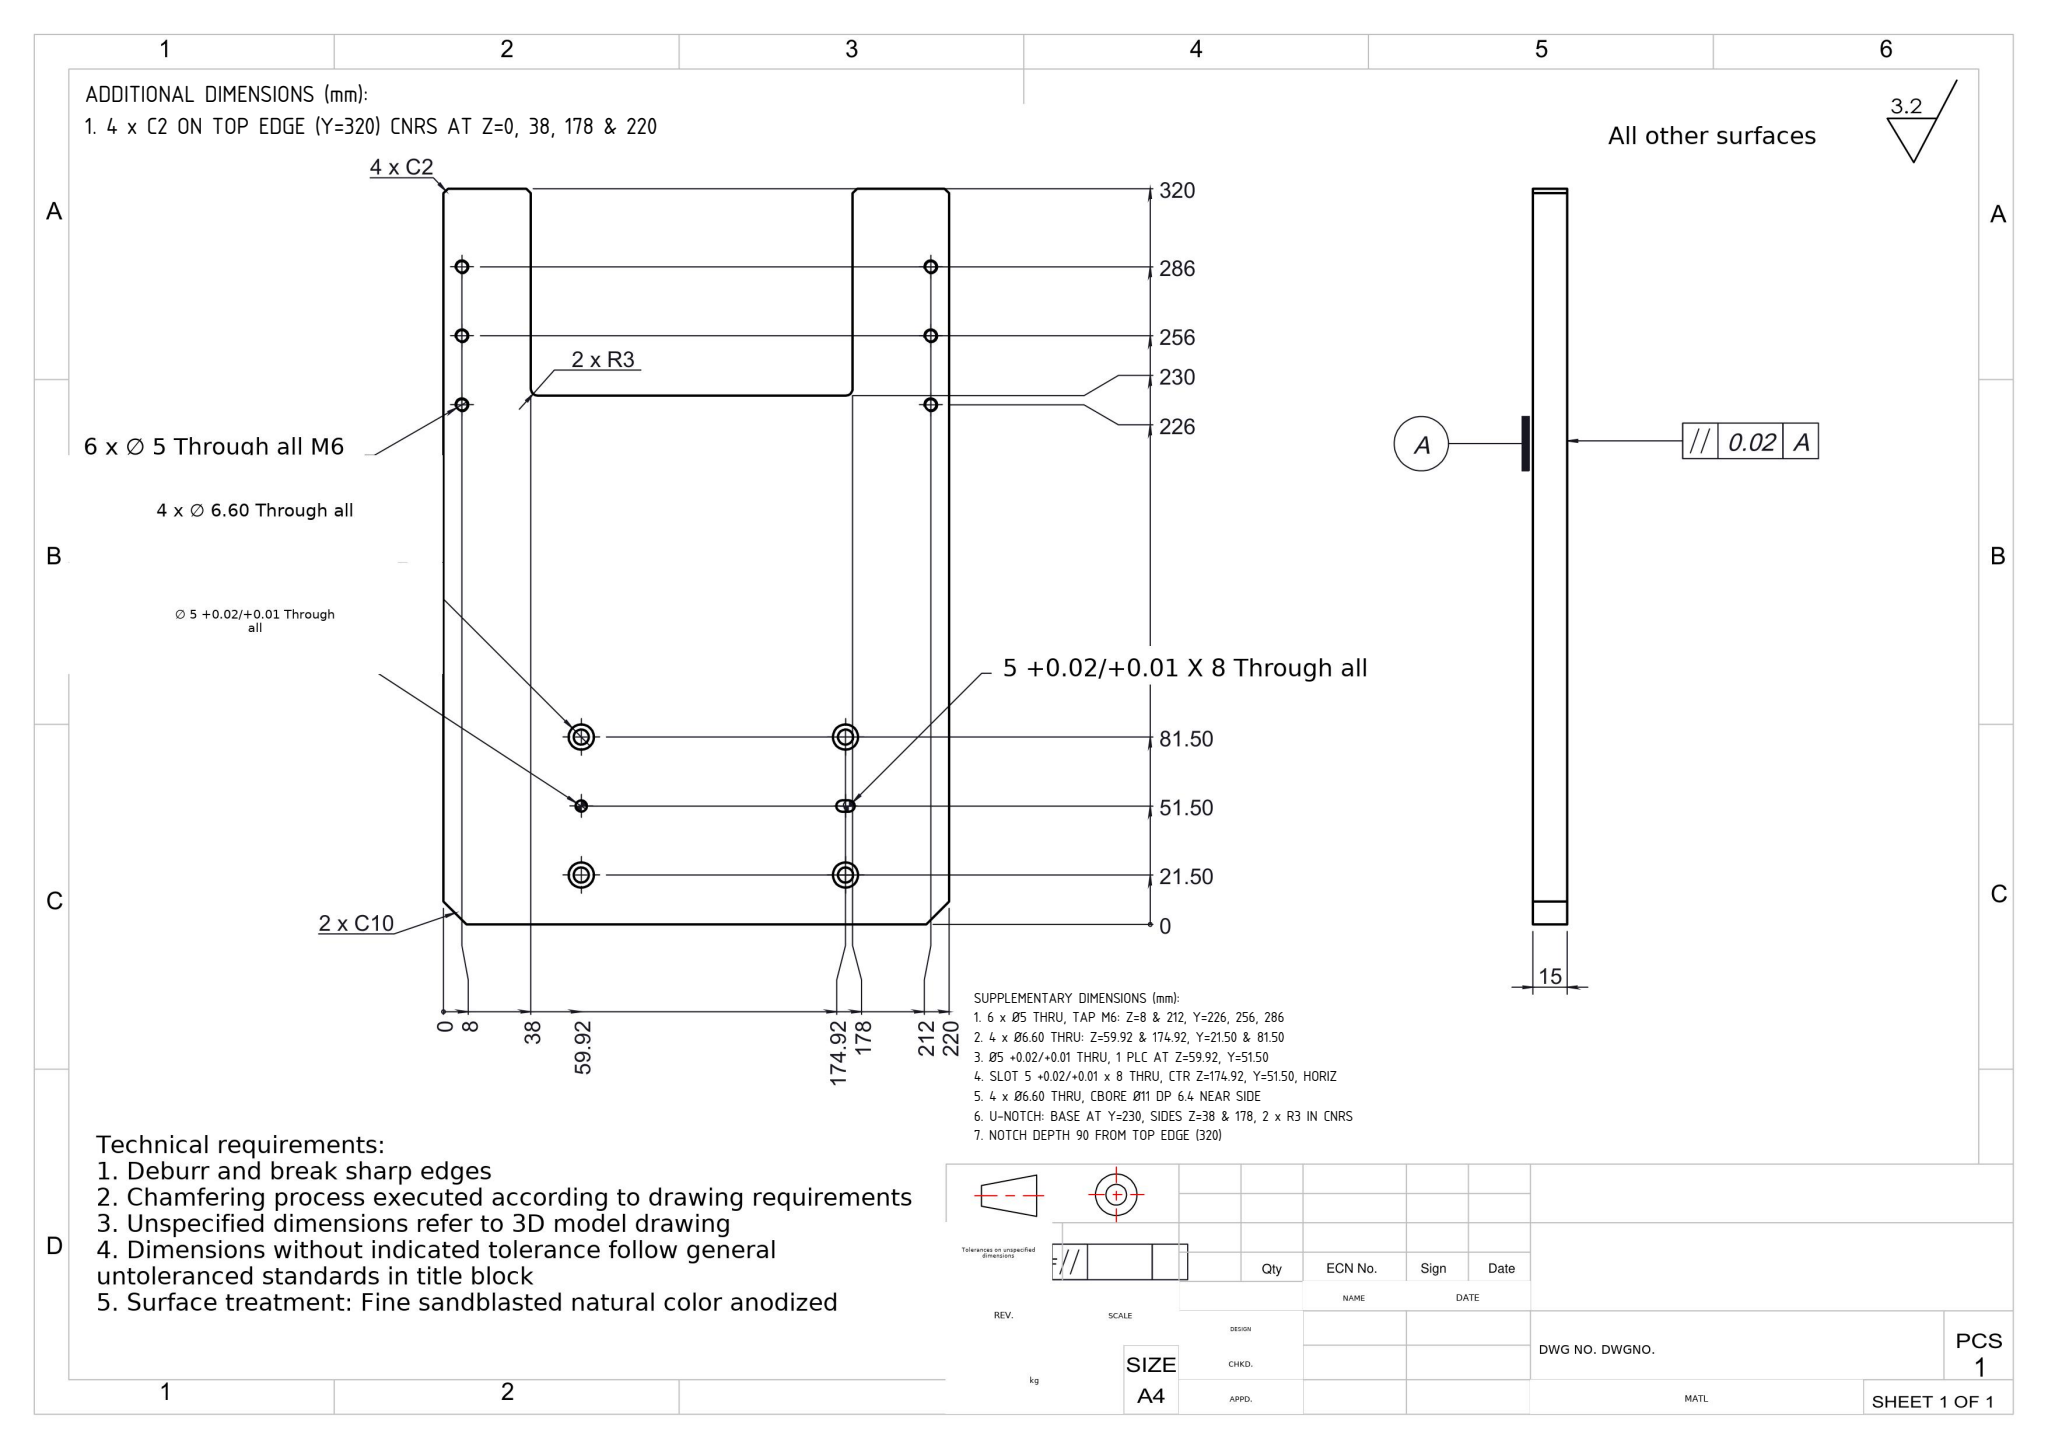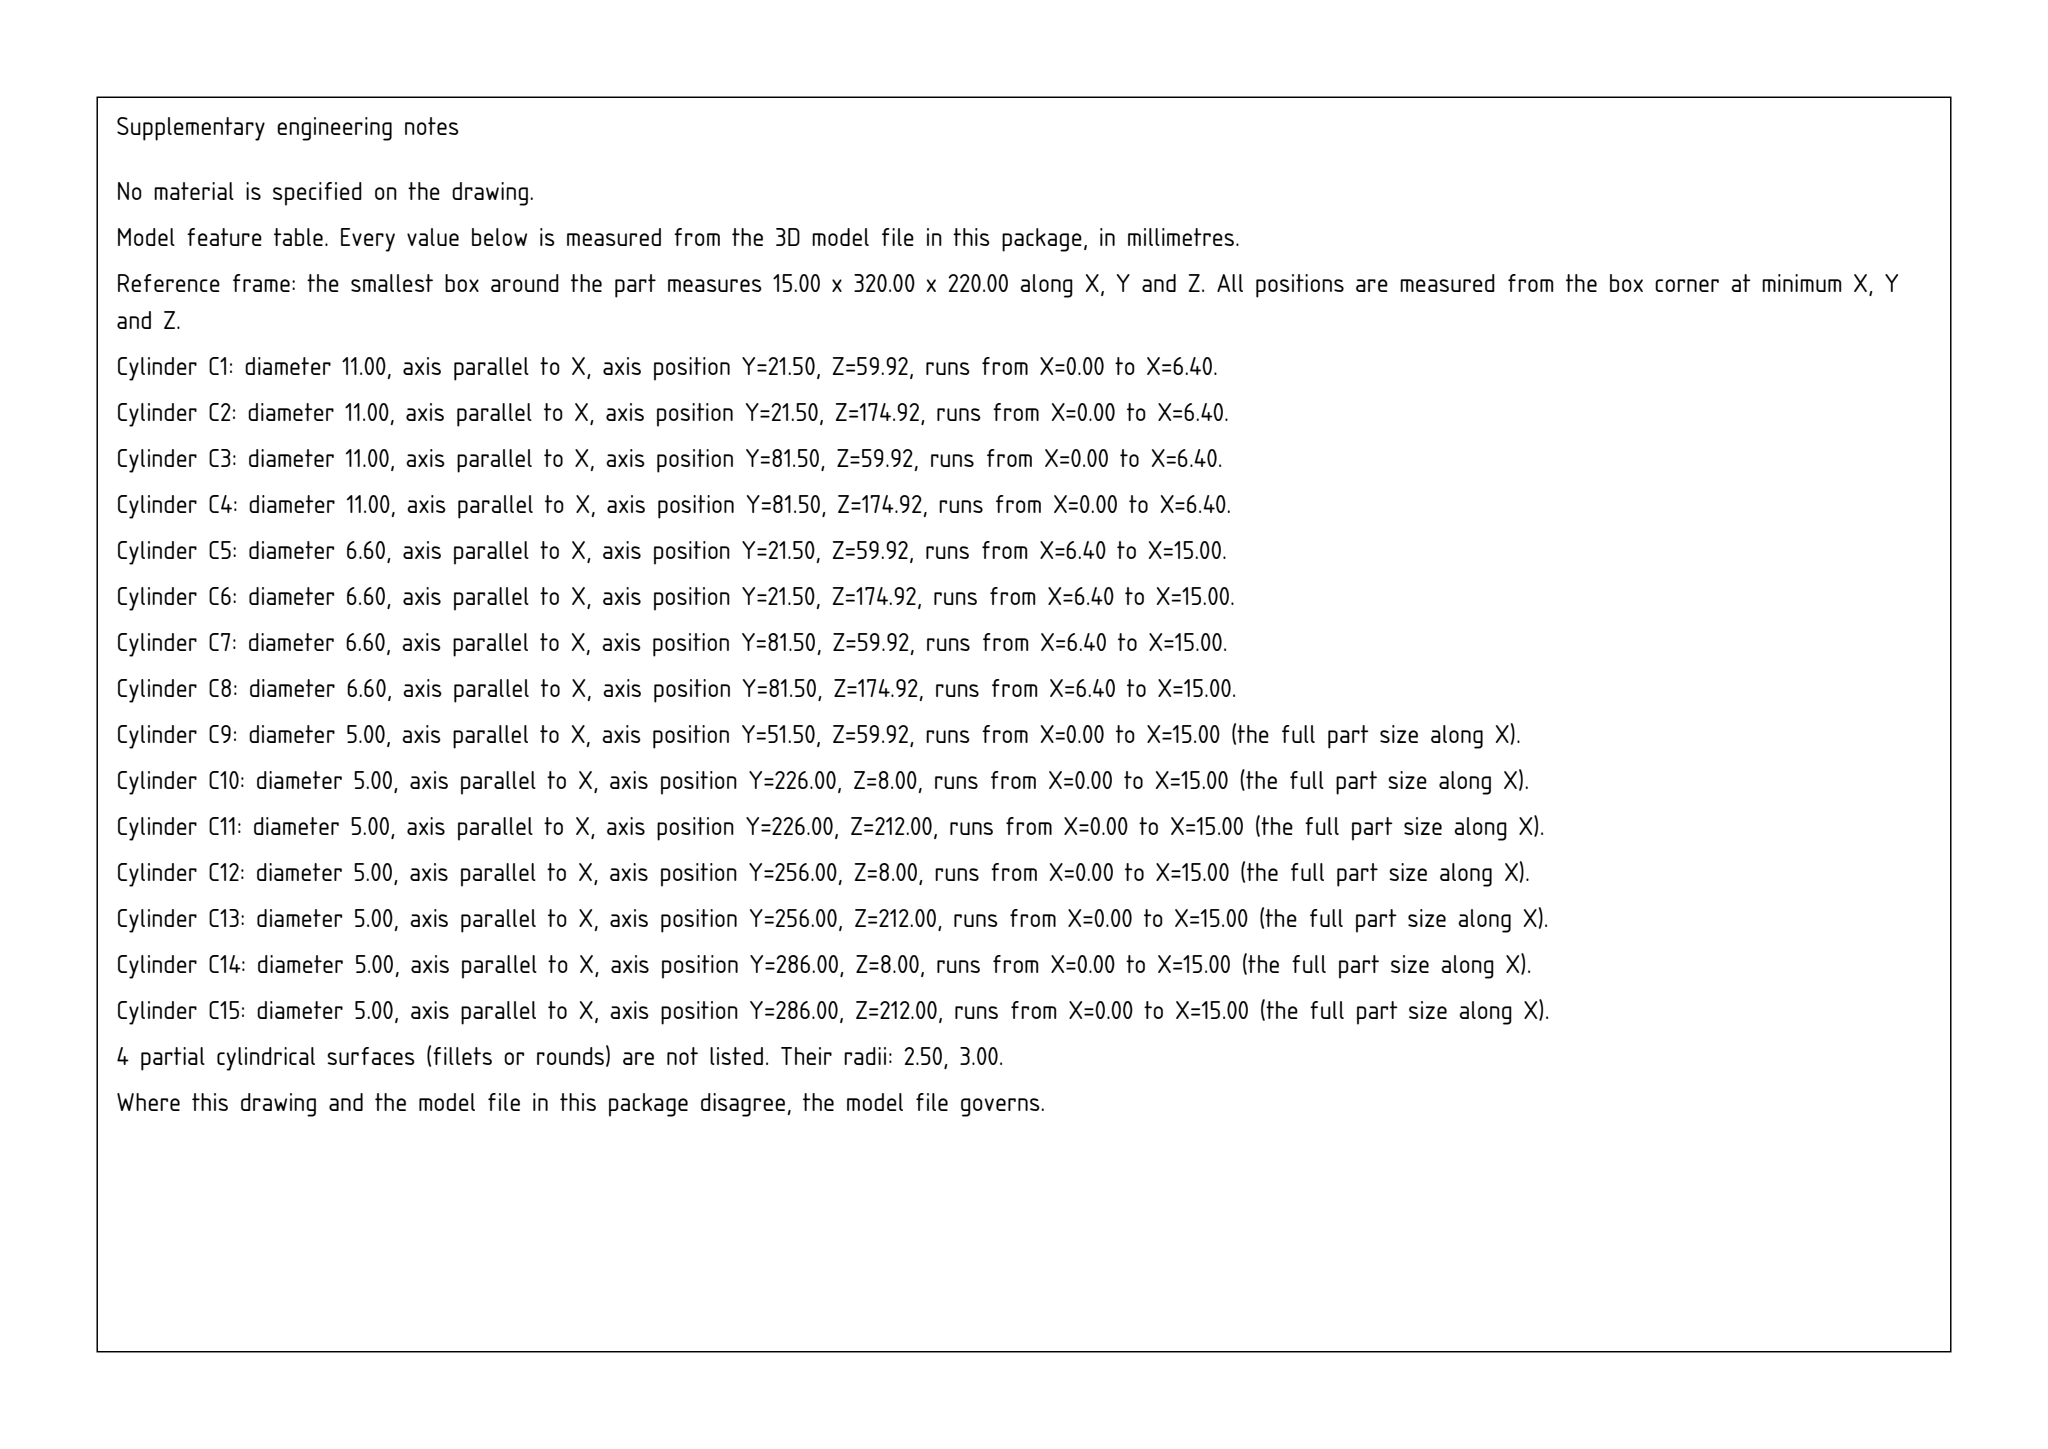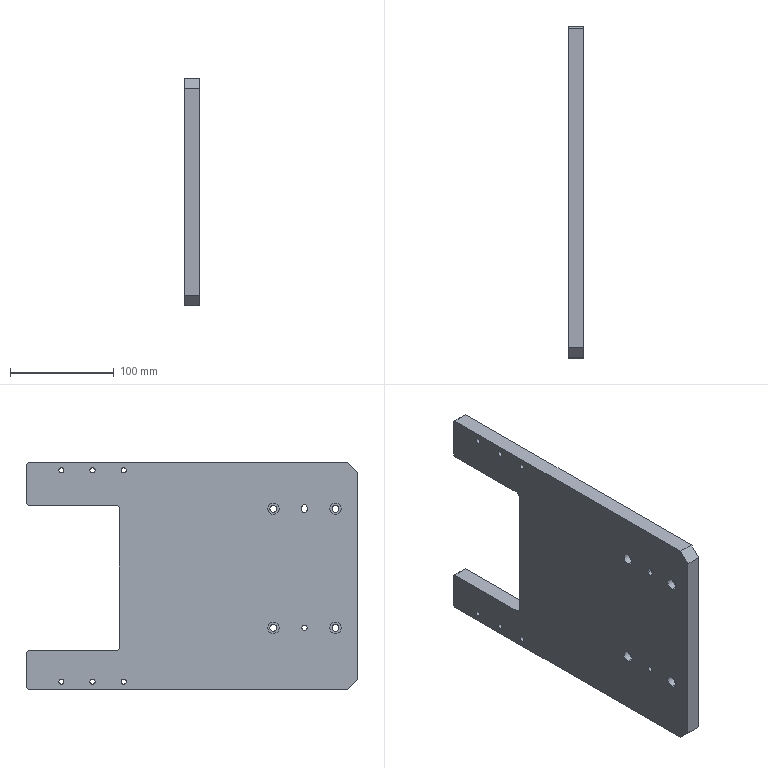Part | SolidWorks | mm | 1 solid | 57 faces | box 15 x 320 x 220 mm | volume 859247 mm3 | cylinder 35 | plane 22 | commonest cylinder face diameters 5 x17 11 x8 6.6 x8 6 x2